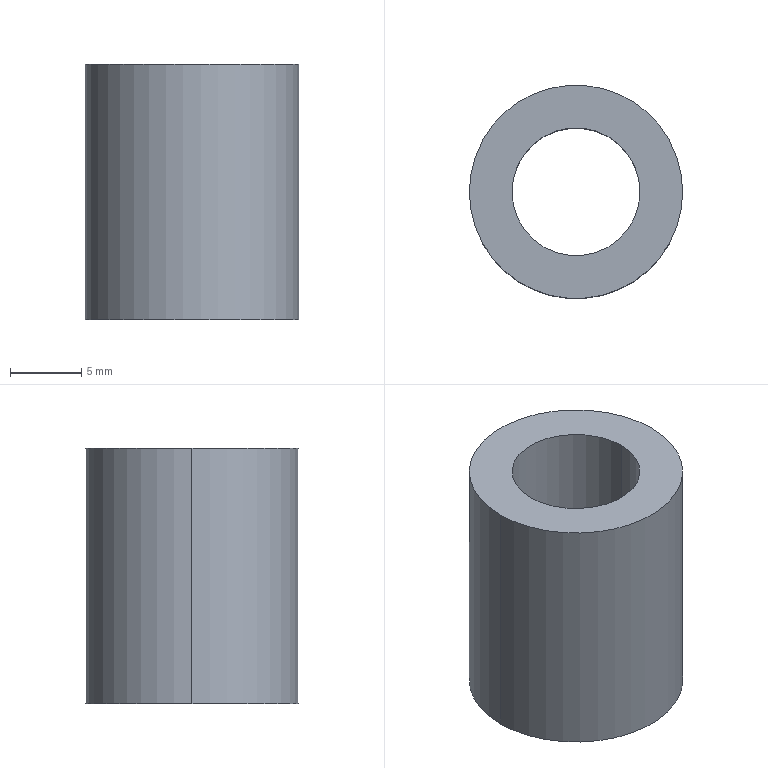Component | SolidWorks | DirectPressureVerticalSeal-1_ThermalInsulationSleeve-1 | 1 solid | 6 faces | box 15 x 15 x 18 mm | volume 2036 mm3 | cylinder 4 | plane 2 | commonest cylinder face diameters 9 x2 15 x2
build123d program:
from build123d import *

# Parameters (mm, degrees)
SKETCH1_W = 3
SKETCH1_H = 18


with BuildPart() as part:
    # Sketch1 → Revolve1 (revolve)
    with BuildSketch(Plane.XZ, mode=Mode.PRIVATE) as revolve1_sk:
        with Locations((6, 0)):
            Rectangle(SKETCH1_W, SKETCH1_H)
    revolve(revolve1_sk.sketch.rotate(Axis((0, 0, 9), (0, 0, -1)), 180), axis=Axis((0, 0, 9), (0, 0, -1)))


solid = part.part

# Placed as in the assembly
solid = solid.moved(Location((-298.746, 331.873, 230.054), (0, 0, 0)))
STEP:
#1=COLOUR_RGB('',0.7922,0.8196,0.9333);
#2=FILL_AREA_STYLE_COLOUR('',#1);
#3=FILL_AREA_STYLE('',(#2));
#4=SURFACE_STYLE_FILL_AREA(#3);
#5=SURFACE_SIDE_STYLE('',(#4));
#6=SURFACE_STYLE_USAGE(.BOTH.,#5);
#7=PRESENTATION_STYLE_ASSIGNMENT((#6));
#8=CARTESIAN_POINT('',(-11.939,13.066,9.412));
#9=VERTEX_POINT('',#8);
#10=CARTESIAN_POINT('',(-11.585,13.066,9.412));
#11=VERTEX_POINT('',#10);
#12=CARTESIAN_POINT('',(-11.762,13.066,9.412));
#13=DIRECTION('',(0.,-0.,-1.));
#14=DIRECTION('',(1.,-0.,0.));
#15=AXIS2_PLACEMENT_3D('',#12,#13,#14);
#16=CIRCLE('',#15,0.1772);
#17=EDGE_CURVE('',#9,#11,#16,.T.);
#18=ORIENTED_EDGE('',*,*,#17,.F.);
#19=CARTESIAN_POINT('',(-11.939,13.066,8.703));
#20=VERTEX_POINT('',#19);
#21=CARTESIAN_POINT('',(-11.939,13.066,9.412));
#22=DIRECTION('',(0.,-0.,-1.));
#23=VECTOR('',#22,39.37);
#24=LINE('',#21,#23);
#25=EDGE_CURVE('',#9,#20,#24,.T.);
#26=ORIENTED_EDGE('',*,*,#25,.T.);
#27=CARTESIAN_POINT('',(-11.585,13.066,8.703));
#28=VERTEX_POINT('',#27);
#29=CARTESIAN_POINT('',(-11.762,13.066,8.703));
#30=DIRECTION('',(0.,-0.,-1.));
#31=DIRECTION('',(1.,-0.,0.));
#32=AXIS2_PLACEMENT_3D('',#29,#30,#31);
#33=CIRCLE('',#32,0.1772);
#34=EDGE_CURVE('',#20,#28,#33,.T.);
#35=ORIENTED_EDGE('',*,*,#34,.T.);
#36=CARTESIAN_POINT('',(-11.585,13.066,9.412));
#37=DIRECTION('',(0.,-0.,-1.));
#38=VECTOR('',#37,39.37);
#39=LINE('',#36,#38);
#40=EDGE_CURVE('',#11,#28,#39,.T.);
#41=ORIENTED_EDGE('',*,*,#40,.F.);
#42=EDGE_LOOP('',(#18,#26,#35,#41));
#43=FACE_OUTER_BOUND('',#42,.T.);
#44=CARTESIAN_POINT('',(-11.762,13.066,9.412));
#45=DIRECTION('',(0.,-0.,-1.));
#46=DIRECTION('',(1.,-0.,0.));
#47=AXIS2_PLACEMENT_3D('',#44,#45,#46);
#48=CYLINDRICAL_SURFACE('',#47,0.1772);
#49=ADVANCED_FACE('',(#43),#48,.F.);
#50=CARTESIAN_POINT('',(-11.466,13.066,9.412));
#51=VERTEX_POINT('',#50);
#52=CARTESIAN_POINT('',(-12.057,13.066,9.412));
#53=VERTEX_POINT('',#52);
#54=CARTESIAN_POINT('',(-11.762,13.066,9.412));
#55=DIRECTION('',(0.,-0.,-1.));
#56=DIRECTION('',(1.,-0.,0.));
#57=AXIS2_PLACEMENT_3D('',#54,#55,#56);
#58=CIRCLE('',#57,0.2953);
#59=EDGE_CURVE('',#51,#53,#58,.T.);
#60=ORIENTED_EDGE('',*,*,#59,.T.);
#61=CARTESIAN_POINT('',(-12.057,13.066,8.703));
#62=VERTEX_POINT('',#61);
#63=CARTESIAN_POINT('',(-12.057,13.066,9.412));
#64=DIRECTION('',(0.,-0.,-1.));
#65=VECTOR('',#64,39.37);
#66=LINE('',#63,#65);
#67=EDGE_CURVE('',#53,#62,#66,.T.);
#68=ORIENTED_EDGE('',*,*,#67,.T.);
#69=CARTESIAN_POINT('',(-11.466,13.066,8.703));
#70=VERTEX_POINT('',#69);
#71=CARTESIAN_POINT('',(-11.762,13.066,8.703));
#72=DIRECTION('',(0.,-0.,-1.));
#73=DIRECTION('',(1.,-0.,0.));
#74=AXIS2_PLACEMENT_3D('',#71,#72,#73);
#75=CIRCLE('',#74,0.2953);
#76=EDGE_CURVE('',#70,#62,#75,.T.);
#77=ORIENTED_EDGE('',*,*,#76,.F.);
#78=CARTESIAN_POINT('',(-11.466,13.066,9.412));
#79=DIRECTION('',(0.,-0.,-1.));
#80=VECTOR('',#79,39.37);
#81=LINE('',#78,#80);
#82=EDGE_CURVE('',#51,#70,#81,.T.);
#83=ORIENTED_EDGE('',*,*,#82,.F.);
#84=EDGE_LOOP('',(#60,#68,#77,#83));
#85=FACE_OUTER_BOUND('',#84,.T.);
#86=CARTESIAN_POINT('',(-11.762,13.066,9.412));
#87=DIRECTION('',(0.,-0.,-1.));
#88=DIRECTION('',(1.,-0.,0.));
#89=AXIS2_PLACEMENT_3D('',#86,#87,#88);
#90=CYLINDRICAL_SURFACE('',#89,0.2953);
#91=ADVANCED_FACE('',(#85),#90,.T.);
#92=ORIENTED_EDGE('',*,*,#67,.F.);
#93=CARTESIAN_POINT('',(-11.762,13.066,9.412));
#94=DIRECTION('',(0.,-0.,-1.));
#95=DIRECTION('',(1.,-0.,0.));
#96=AXIS2_PLACEMENT_3D('',#93,#94,#95);
#97=CIRCLE('',#96,0.2953);
#98=EDGE_CURVE('',#53,#51,#97,.T.);
#99=ORIENTED_EDGE('',*,*,#98,.T.);
#100=ORIENTED_EDGE('',*,*,#82,.T.);
#101=CARTESIAN_POINT('',(-11.762,13.066,8.703));
#102=DIRECTION('',(0.,-0.,-1.));
#103=DIRECTION('',(1.,-0.,0.));
#104=AXIS2_PLACEMENT_3D('',#101,#102,#103);
#105=CIRCLE('',#104,0.2953);
#106=EDGE_CURVE('',#62,#70,#105,.T.);
#107=ORIENTED_EDGE('',*,*,#106,.F.);
#108=EDGE_LOOP('',(#92,#99,#100,#107));
#109=FACE_OUTER_BOUND('',#108,.T.);
#110=CARTESIAN_POINT('',(-11.762,13.066,9.412));
#111=DIRECTION('',(0.,-0.,-1.));
#112=DIRECTION('',(1.,-0.,0.));
#113=AXIS2_PLACEMENT_3D('',#110,#111,#112);
#114=CYLINDRICAL_SURFACE('',#113,0.2953);
#115=ADVANCED_FACE('',(#109),#114,.T.);
#116=CARTESIAN_POINT('',(-11.762,13.066,9.412));
#117=DIRECTION('',(0.,-0.,-1.));
#118=DIRECTION('',(1.,-0.,0.));
#119=AXIS2_PLACEMENT_3D('',#116,#117,#118);
#120=CIRCLE('',#119,0.1772);
#121=EDGE_CURVE('',#11,#9,#120,.T.);
#122=ORIENTED_EDGE('',*,*,#121,.T.);
#123=ORIENTED_EDGE('',*,*,#17,.T.);
#124=EDGE_LOOP('',(#122,#123));
#125=FACE_BOUND('',#124,.T.);
#126=ORIENTED_EDGE('',*,*,#59,.F.);
#127=ORIENTED_EDGE('',*,*,#98,.F.);
#128=EDGE_LOOP('',(#126,#127));
#129=FACE_OUTER_BOUND('',#128,.T.);
#130=CARTESIAN_POINT('',(-12.057,13.066,9.412));
#131=DIRECTION('',(-0.,0.,1.));
#132=DIRECTION('',(-1.,0.,-0.));
#133=AXIS2_PLACEMENT_3D('',#130,#131,#132);
#134=PLANE('',#133);
#135=ADVANCED_FACE('',(#125,#129),#134,.T.);
#136=ORIENTED_EDGE('',*,*,#25,.F.);
#137=ORIENTED_EDGE('',*,*,#121,.F.);
#138=ORIENTED_EDGE('',*,*,#40,.T.);
#139=CARTESIAN_POINT('',(-11.762,13.066,8.703));
#140=DIRECTION('',(0.,-0.,-1.));
#141=DIRECTION('',(1.,-0.,0.));
#142=AXIS2_PLACEMENT_3D('',#139,#140,#141);
#143=CIRCLE('',#142,0.1772);
#144=EDGE_CURVE('',#28,#20,#143,.T.);
#145=ORIENTED_EDGE('',*,*,#144,.T.);
#146=EDGE_LOOP('',(#136,#137,#138,#145));
#147=FACE_OUTER_BOUND('',#146,.T.);
#148=CARTESIAN_POINT('',(-11.762,13.066,9.412));
#149=DIRECTION('',(0.,-0.,-1.));
#150=DIRECTION('',(1.,-0.,0.));
#151=AXIS2_PLACEMENT_3D('',#148,#149,#150);
#152=CYLINDRICAL_SURFACE('',#151,0.1772);
#153=ADVANCED_FACE('',(#147),#152,.F.);
#154=ORIENTED_EDGE('',*,*,#76,.T.);
#155=ORIENTED_EDGE('',*,*,#106,.T.);
#156=EDGE_LOOP('',(#154,#155));
#157=FACE_OUTER_BOUND('',#156,.T.);
#158=ORIENTED_EDGE('',*,*,#144,.F.);
#159=ORIENTED_EDGE('',*,*,#34,.F.);
#160=EDGE_LOOP('',(#158,#159));
#161=FACE_BOUND('',#160,.T.);
#162=CARTESIAN_POINT('',(-11.939,13.066,8.703));
#163=DIRECTION('',(0.,-0.,-1.));
#164=DIRECTION('',(1.,-0.,0.));
#165=AXIS2_PLACEMENT_3D('',#162,#163,#164);
#166=PLANE('',#165);
#167=ADVANCED_FACE('',(#157,#161),#166,.T.);
#168=CLOSED_SHELL('',(#49,#91,#115,#135,#153,#167));
#169=MANIFOLD_SOLID_BREP('',#168);
#170=STYLED_ITEM('',(#7),#169);
#171=(LENGTH_UNIT()NAMED_UNIT(*)SI_UNIT($,.METRE.));
#172=LENGTH_MEASURE_WITH_UNIT(LENGTH_MEASURE(0.0254),#171);
#173=DIMENSIONAL_EXPONENTS(1.,0.,0.,0.,0.,0.,0.);
#174=(CONVERSION_BASED_UNIT('',#172)LENGTH_UNIT()NAMED_UNIT(#173));
#175=UNCERTAINTY_MEASURE_WITH_UNIT(LENGTH_MEASURE(0.00001),#174,'','');
#176=(NAMED_UNIT(*)PLANE_ANGLE_UNIT()SI_UNIT($,.RADIAN.));
#177=(NAMED_UNIT(*)SI_UNIT($,.STERADIAN.)SOLID_ANGLE_UNIT());
#178=(GEOMETRIC_REPRESENTATION_CONTEXT(3)GLOBAL_UNCERTAINTY_ASSIGNED_CONTEXT((#175))GLOBAL_UNIT_ASSIGNED_CONTEXT((#174,#176,#177))REPRESENTATION_CONTEXT('',''));
#179=MECHANICAL_DESIGN_GEOMETRIC_PRESENTATION_REPRESENTATION('',(#170),#178);
#180=CARTESIAN_POINT('',(0.,0.,0.));
#181=DIRECTION('',(0.,0.,1.));
#182=DIRECTION('',(1.,0.,0.));
#183=AXIS2_PLACEMENT_3D('',#180,#181,#182);
#184=(LENGTH_UNIT()NAMED_UNIT(*)SI_UNIT($,.METRE.));
#185=LENGTH_MEASURE_WITH_UNIT(LENGTH_MEASURE(0.0254),#184);
#186=DIMENSIONAL_EXPONENTS(1.,0.,0.,0.,0.,0.,0.);
#187=(CONVERSION_BASED_UNIT('',#185)LENGTH_UNIT()NAMED_UNIT(#186));
#188=UNCERTAINTY_MEASURE_WITH_UNIT(LENGTH_MEASURE(0.00001),#187,'','');
#189=(NAMED_UNIT(*)PLANE_ANGLE_UNIT()SI_UNIT($,.RADIAN.));
#190=(NAMED_UNIT(*)SI_UNIT($,.STERADIAN.)SOLID_ANGLE_UNIT());
#191=(GEOMETRIC_REPRESENTATION_CONTEXT(3)GLOBAL_UNCERTAINTY_ASSIGNED_CONTEXT((#188))GLOBAL_UNIT_ASSIGNED_CONTEXT((#187,#189,#190))REPRESENTATION_CONTEXT('',''));
#192=ADVANCED_BREP_SHAPE_REPRESENTATION('',(#169,#183),#191);
#193=PRESENTATION_LAYER_ASSIGNMENT('','',(#170));